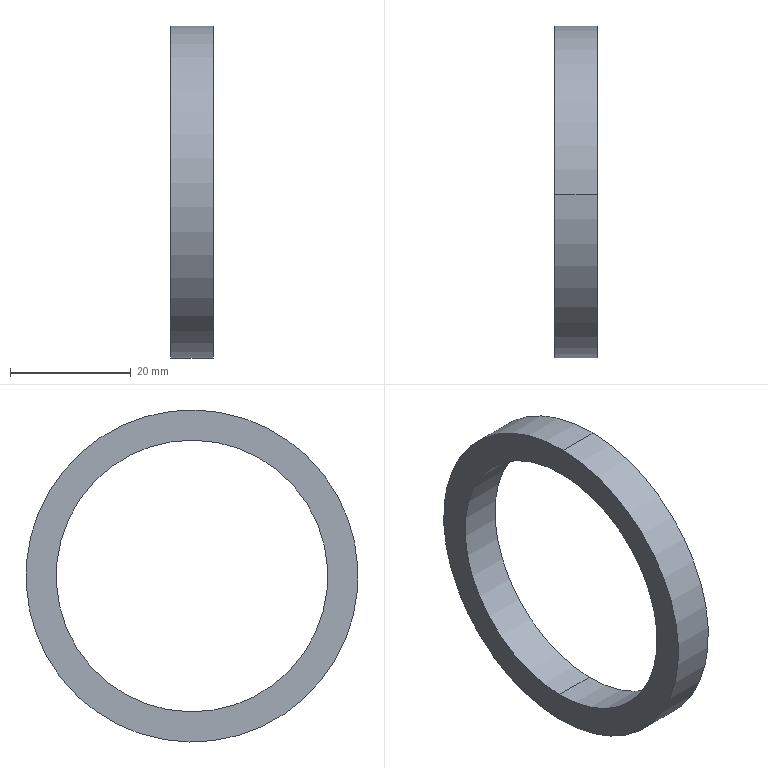Component | SolidWorks | 216InnerTubeAssembly-1_BearingSpacer2-1 | 1 solid | 6 faces | box 7 x 55 x 55 mm | volume 5498 mm3 | cylinder 4 | plane 2 | commonest cylinder face diameters 45 x2 55 x2 | material Alloy Steel
build123d program:
from build123d import *


with BuildPart() as part:
    # Model → Revolve1 (revolve)
    with BuildSketch(Plane.XY, mode=Mode.PRIVATE) as revolve1_sk:
        Polygon((7, 22.5), (7, 27.5), (2, 27.5), (0, 27.5), (0, 22.5), align=None)
    revolve(revolve1_sk.sketch.rotate(Axis((0, 0, 0), (1, 0, 0)), 90), axis=Axis((0, 0, 0), (1, 0, 0)))


solid = part.part

# Placed as in the assembly
solid = solid.moved(Location((905.278, 0, 0), (0, 0, 0)))
STEP:
#1=COLOUR_RGB('',0.7922,0.8196,0.9333);
#2=FILL_AREA_STYLE_COLOUR('',#1);
#3=FILL_AREA_STYLE('',(#2));
#4=SURFACE_STYLE_FILL_AREA(#3);
#5=SURFACE_SIDE_STYLE('',(#4));
#6=SURFACE_STYLE_USAGE(.BOTH.,#5);
#7=PRESENTATION_STYLE_ASSIGNMENT((#6));
#8=CARTESIAN_POINT('',(35.916,0.01591,-0.8857));
#9=VERTEX_POINT('',#8);
#10=CARTESIAN_POINT('',(35.916,-0.01591,0.8857));
#11=VERTEX_POINT('',#10);
#12=CARTESIAN_POINT('',(35.916,-0.,0.));
#13=DIRECTION('',(-1.,-0.,0.));
#14=DIRECTION('',(0.,-0.01796,0.9998));
#15=AXIS2_PLACEMENT_3D('',#12,#13,#14);
#16=CIRCLE('',#15,0.8858);
#17=EDGE_CURVE('',#9,#11,#16,.T.);
#18=ORIENTED_EDGE('',*,*,#17,.F.);
#19=CARTESIAN_POINT('',(35.641,0.01591,-0.8857));
#20=VERTEX_POINT('',#19);
#21=CARTESIAN_POINT('',(35.641,0.01591,-0.8857));
#22=DIRECTION('',(-1.,-0.,0.));
#23=VECTOR('',#22,39.37);
#24=LINE('',#21,#23);
#25=EDGE_CURVE('',#9,#20,#24,.T.);
#26=ORIENTED_EDGE('',*,*,#25,.T.);
#27=CARTESIAN_POINT('',(35.641,-0.01591,0.8857));
#28=VERTEX_POINT('',#27);
#29=CARTESIAN_POINT('',(35.641,-0.,0.));
#30=DIRECTION('',(-1.,-0.,0.));
#31=DIRECTION('',(0.,-0.01796,0.9998));
#32=AXIS2_PLACEMENT_3D('',#29,#30,#31);
#33=CIRCLE('',#32,0.8858);
#34=EDGE_CURVE('',#20,#28,#33,.T.);
#35=ORIENTED_EDGE('',*,*,#34,.T.);
#36=CARTESIAN_POINT('',(35.641,-0.01591,0.8857));
#37=DIRECTION('',(-1.,-0.,0.));
#38=VECTOR('',#37,39.37);
#39=LINE('',#36,#38);
#40=EDGE_CURVE('',#11,#28,#39,.T.);
#41=ORIENTED_EDGE('',*,*,#40,.F.);
#42=EDGE_LOOP('',(#18,#26,#35,#41));
#43=FACE_OUTER_BOUND('',#42,.T.);
#44=CARTESIAN_POINT('',(35.641,-0.,0.));
#45=DIRECTION('',(-1.,-0.,0.));
#46=DIRECTION('',(0.,-0.01796,0.9998));
#47=AXIS2_PLACEMENT_3D('',#44,#45,#46);
#48=CYLINDRICAL_SURFACE('',#47,0.8858);
#49=ADVANCED_FACE('',(#43),#48,.F.);
#50=CARTESIAN_POINT('',(35.916,-0.01944,1.083));
#51=VERTEX_POINT('',#50);
#52=CARTESIAN_POINT('',(35.916,0.01944,-1.083));
#53=VERTEX_POINT('',#52);
#54=CARTESIAN_POINT('',(35.916,-0.,0.));
#55=DIRECTION('',(-1.,-0.,0.));
#56=DIRECTION('',(0.,-0.01796,0.9998));
#57=AXIS2_PLACEMENT_3D('',#54,#55,#56);
#58=CIRCLE('',#57,1.083);
#59=EDGE_CURVE('',#51,#53,#58,.T.);
#60=ORIENTED_EDGE('',*,*,#59,.T.);
#61=CARTESIAN_POINT('',(35.641,0.01944,-1.083));
#62=VERTEX_POINT('',#61);
#63=CARTESIAN_POINT('',(35.641,0.01944,-1.083));
#64=DIRECTION('',(-1.,-0.,0.));
#65=VECTOR('',#64,39.37);
#66=LINE('',#63,#65);
#67=EDGE_CURVE('',#53,#62,#66,.T.);
#68=ORIENTED_EDGE('',*,*,#67,.T.);
#69=CARTESIAN_POINT('',(35.641,-0.01944,1.083));
#70=VERTEX_POINT('',#69);
#71=CARTESIAN_POINT('',(35.641,-0.,0.));
#72=DIRECTION('',(-1.,-0.,0.));
#73=DIRECTION('',(0.,-0.01796,0.9998));
#74=AXIS2_PLACEMENT_3D('',#71,#72,#73);
#75=CIRCLE('',#74,1.083);
#76=EDGE_CURVE('',#70,#62,#75,.T.);
#77=ORIENTED_EDGE('',*,*,#76,.F.);
#78=CARTESIAN_POINT('',(35.641,-0.01944,1.083));
#79=DIRECTION('',(-1.,-0.,0.));
#80=VECTOR('',#79,39.37);
#81=LINE('',#78,#80);
#82=EDGE_CURVE('',#51,#70,#81,.T.);
#83=ORIENTED_EDGE('',*,*,#82,.F.);
#84=EDGE_LOOP('',(#60,#68,#77,#83));
#85=FACE_OUTER_BOUND('',#84,.T.);
#86=CARTESIAN_POINT('',(35.641,-0.,0.));
#87=DIRECTION('',(-1.,-0.,0.));
#88=DIRECTION('',(0.,-0.01796,0.9998));
#89=AXIS2_PLACEMENT_3D('',#86,#87,#88);
#90=CYLINDRICAL_SURFACE('',#89,1.083);
#91=ADVANCED_FACE('',(#85),#90,.T.);
#92=ORIENTED_EDGE('',*,*,#67,.F.);
#93=CARTESIAN_POINT('',(35.916,-0.,0.));
#94=DIRECTION('',(-1.,-0.,0.));
#95=DIRECTION('',(0.,-0.01796,0.9998));
#96=AXIS2_PLACEMENT_3D('',#93,#94,#95);
#97=CIRCLE('',#96,1.083);
#98=EDGE_CURVE('',#53,#51,#97,.T.);
#99=ORIENTED_EDGE('',*,*,#98,.T.);
#100=ORIENTED_EDGE('',*,*,#82,.T.);
#101=CARTESIAN_POINT('',(35.641,-0.,0.));
#102=DIRECTION('',(-1.,-0.,0.));
#103=DIRECTION('',(0.,-0.01796,0.9998));
#104=AXIS2_PLACEMENT_3D('',#101,#102,#103);
#105=CIRCLE('',#104,1.083);
#106=EDGE_CURVE('',#62,#70,#105,.T.);
#107=ORIENTED_EDGE('',*,*,#106,.F.);
#108=EDGE_LOOP('',(#92,#99,#100,#107));
#109=FACE_OUTER_BOUND('',#108,.T.);
#110=CARTESIAN_POINT('',(35.641,-0.,0.));
#111=DIRECTION('',(-1.,-0.,0.));
#112=DIRECTION('',(0.,-0.01796,0.9998));
#113=AXIS2_PLACEMENT_3D('',#110,#111,#112);
#114=CYLINDRICAL_SURFACE('',#113,1.083);
#115=ADVANCED_FACE('',(#109),#114,.T.);
#116=CARTESIAN_POINT('',(35.641,-0.,0.));
#117=DIRECTION('',(-1.,-0.,0.));
#118=DIRECTION('',(0.,-0.01796,0.9998));
#119=AXIS2_PLACEMENT_3D('',#116,#117,#118);
#120=CIRCLE('',#119,0.8858);
#121=EDGE_CURVE('',#28,#20,#120,.T.);
#122=ORIENTED_EDGE('',*,*,#121,.F.);
#123=ORIENTED_EDGE('',*,*,#34,.F.);
#124=EDGE_LOOP('',(#122,#123));
#125=FACE_BOUND('',#124,.T.);
#126=ORIENTED_EDGE('',*,*,#76,.T.);
#127=ORIENTED_EDGE('',*,*,#106,.T.);
#128=EDGE_LOOP('',(#126,#127));
#129=FACE_OUTER_BOUND('',#128,.T.);
#130=CARTESIAN_POINT('',(35.641,-0.,0.));
#131=DIRECTION('',(1.,0.,-0.));
#132=DIRECTION('',(-0.,0.01796,-0.9998));
#133=AXIS2_PLACEMENT_3D('',#130,#131,#132);
#134=PLANE('',#133);
#135=ADVANCED_FACE('',(#125,#129),#134,.F.);
#136=ORIENTED_EDGE('',*,*,#25,.F.);
#137=CARTESIAN_POINT('',(35.916,-0.,0.));
#138=DIRECTION('',(-1.,-0.,0.));
#139=DIRECTION('',(0.,-0.01796,0.9998));
#140=AXIS2_PLACEMENT_3D('',#137,#138,#139);
#141=CIRCLE('',#140,0.8858);
#142=EDGE_CURVE('',#11,#9,#141,.T.);
#143=ORIENTED_EDGE('',*,*,#142,.F.);
#144=ORIENTED_EDGE('',*,*,#40,.T.);
#145=ORIENTED_EDGE('',*,*,#121,.T.);
#146=EDGE_LOOP('',(#136,#143,#144,#145));
#147=FACE_OUTER_BOUND('',#146,.T.);
#148=CARTESIAN_POINT('',(35.641,-0.,0.));
#149=DIRECTION('',(-1.,-0.,0.));
#150=DIRECTION('',(0.,-0.01796,0.9998));
#151=AXIS2_PLACEMENT_3D('',#148,#149,#150);
#152=CYLINDRICAL_SURFACE('',#151,0.8858);
#153=ADVANCED_FACE('',(#147),#152,.F.);
#154=ORIENTED_EDGE('',*,*,#59,.F.);
#155=ORIENTED_EDGE('',*,*,#98,.F.);
#156=EDGE_LOOP('',(#154,#155));
#157=FACE_OUTER_BOUND('',#156,.T.);
#158=ORIENTED_EDGE('',*,*,#142,.T.);
#159=ORIENTED_EDGE('',*,*,#17,.T.);
#160=EDGE_LOOP('',(#158,#159));
#161=FACE_BOUND('',#160,.T.);
#162=CARTESIAN_POINT('',(35.916,-0.,0.));
#163=DIRECTION('',(-1.,-0.,0.));
#164=DIRECTION('',(0.,-0.01796,0.9998));
#165=AXIS2_PLACEMENT_3D('',#162,#163,#164);
#166=PLANE('',#165);
#167=ADVANCED_FACE('',(#157,#161),#166,.F.);
#168=CLOSED_SHELL('',(#49,#91,#115,#135,#153,#167));
#169=MANIFOLD_SOLID_BREP('',#168);
#170=STYLED_ITEM('',(#7),#169);
#171=(LENGTH_UNIT()NAMED_UNIT(*)SI_UNIT($,.METRE.));
#172=LENGTH_MEASURE_WITH_UNIT(LENGTH_MEASURE(0.0254),#171);
#173=DIMENSIONAL_EXPONENTS(1.,0.,0.,0.,0.,0.,0.);
#174=(CONVERSION_BASED_UNIT('',#172)LENGTH_UNIT()NAMED_UNIT(#173));
#175=UNCERTAINTY_MEASURE_WITH_UNIT(LENGTH_MEASURE(0.00001),#174,'','');
#176=(NAMED_UNIT(*)PLANE_ANGLE_UNIT()SI_UNIT($,.RADIAN.));
#177=(NAMED_UNIT(*)SI_UNIT($,.STERADIAN.)SOLID_ANGLE_UNIT());
#178=(GEOMETRIC_REPRESENTATION_CONTEXT(3)GLOBAL_UNCERTAINTY_ASSIGNED_CONTEXT((#175))GLOBAL_UNIT_ASSIGNED_CONTEXT((#174,#176,#177))REPRESENTATION_CONTEXT('',''));
#179=MECHANICAL_DESIGN_GEOMETRIC_PRESENTATION_REPRESENTATION('',(#170),#178);
#180=PRESENTATION_LAYER_ASSIGNMENT('','',(#170));
#181=CARTESIAN_POINT('',(0.,0.,0.));
#182=DIRECTION('',(0.,0.,1.));
#183=DIRECTION('',(1.,0.,0.));
#184=AXIS2_PLACEMENT_3D('',#181,#182,#183);
#185=(LENGTH_UNIT()NAMED_UNIT(*)SI_UNIT($,.METRE.));
#186=LENGTH_MEASURE_WITH_UNIT(LENGTH_MEASURE(0.0254),#185);
#187=DIMENSIONAL_EXPONENTS(1.,0.,0.,0.,0.,0.,0.);
#188=(CONVERSION_BASED_UNIT('',#186)LENGTH_UNIT()NAMED_UNIT(#187));
#189=UNCERTAINTY_MEASURE_WITH_UNIT(LENGTH_MEASURE(0.00001),#188,'','');
#190=(NAMED_UNIT(*)PLANE_ANGLE_UNIT()SI_UNIT($,.RADIAN.));
#191=(NAMED_UNIT(*)SI_UNIT($,.STERADIAN.)SOLID_ANGLE_UNIT());
#192=(GEOMETRIC_REPRESENTATION_CONTEXT(3)GLOBAL_UNCERTAINTY_ASSIGNED_CONTEXT((#189))GLOBAL_UNIT_ASSIGNED_CONTEXT((#188,#190,#191))REPRESENTATION_CONTEXT('',''));
#193=ADVANCED_BREP_SHAPE_REPRESENTATION('',(#169,#184),#192);